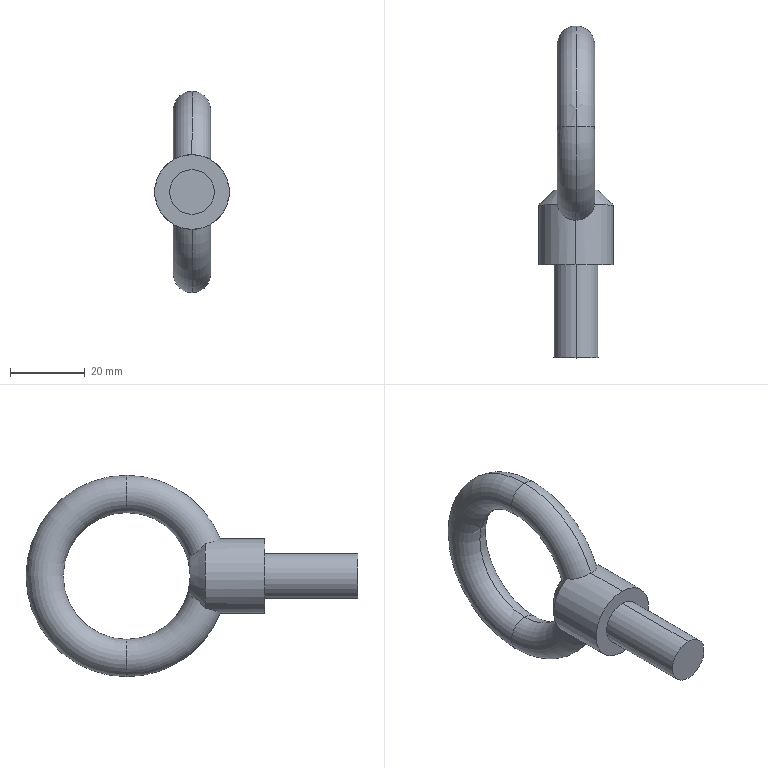Component | SolidWorks | LiftingRingM12-1 | 1 solid | 16 faces | box 20 x 89 x 54 mm | volume 18196 mm3 | torus 6 | cylinder 4 | plane 4 | cone 2 | commonest cylinder face diameters 12 x2 20 x2
STEP:
#1=COLOUR_RGB('',0.7922,0.8196,0.9333);
#2=FILL_AREA_STYLE_COLOUR('',#1);
#3=FILL_AREA_STYLE('',(#2));
#4=SURFACE_STYLE_FILL_AREA(#3);
#5=SURFACE_SIDE_STYLE('',(#4));
#6=SURFACE_STYLE_USAGE(.BOTH.,#5);
#7=PRESENTATION_STYLE_ASSIGNMENT((#6));
#8=CARTESIAN_POINT('',(10.903,79.349,13.168));
#9=VERTEX_POINT('',#8);
#10=CARTESIAN_POINT('',(10.903,79.349,12.775));
#11=VERTEX_POINT('',#10);
#12=CARTESIAN_POINT('',(10.903,79.349,12.971));
#13=DIRECTION('',(0.,1.,0.));
#14=DIRECTION('',(0.,0.,1.));
#15=AXIS2_PLACEMENT_3D('',#12,#13,#14);
#16=CIRCLE('',#15,0.1969);
#17=EDGE_CURVE('',#9,#11,#16,.T.);
#18=ORIENTED_EDGE('',*,*,#17,.F.);
#19=CARTESIAN_POINT('',(10.903,78.361,12.499));
#20=VERTEX_POINT('',#19);
#21=CARTESIAN_POINT('',(10.903,79.349,12.105));
#22=DIRECTION('',(1.,0.,-0.));
#23=DIRECTION('',(0.,0.,-1.));
#24=AXIS2_PLACEMENT_3D('',#21,#22,#23);
#25=CIRCLE('',#24,1.063);
#26=EDGE_CURVE('',#9,#20,#25,.T.);
#27=ORIENTED_EDGE('',*,*,#26,.T.);
#28=CARTESIAN_POINT('',(11.098,78.522,12.447));
#29=VERTEX_POINT('',#28);
#30=CARTESIAN_POINT('',(10.903,78.361,12.499));
#31=CARTESIAN_POINT('',(10.915,78.361,12.499));
#32=CARTESIAN_POINT('',(10.927,78.362,12.498));
#33=CARTESIAN_POINT('',(10.95,78.366,12.496));
#34=CARTESIAN_POINT('',(10.961,78.369,12.495));
#35=CARTESIAN_POINT('',(10.983,78.376,12.491));
#36=CARTESIAN_POINT('',(10.994,78.381,12.489));
#37=CARTESIAN_POINT('',(11.014,78.392,12.483));
#38=CARTESIAN_POINT('',(11.024,78.398,12.48));
#39=CARTESIAN_POINT('',(11.041,78.412,12.474));
#40=CARTESIAN_POINT('',(11.049,78.42,12.471));
#41=CARTESIAN_POINT('',(11.064,78.437,12.465));
#42=CARTESIAN_POINT('',(11.071,78.446,12.462));
#43=CARTESIAN_POINT('',(11.079,78.461,12.458));
#44=CARTESIAN_POINT('',(11.082,78.466,12.456));
#45=CARTESIAN_POINT('',(11.086,78.477,12.454));
#46=CARTESIAN_POINT('',(11.088,78.483,12.453));
#47=CARTESIAN_POINT('',(11.094,78.499,12.45));
#48=CARTESIAN_POINT('',(11.096,78.51,12.448));
#49=CARTESIAN_POINT('',(11.098,78.522,12.447));
#50=B_SPLINE_CURVE_WITH_KNOTS('',3,(#30,#31,#32,#33,#34,#35,#36,#37,#38,#39,#40,#41,#42,#43,#44,#45,#46,#47,#48,#49),.UNSPECIFIED.,.F.,.F.,(4,2,2,2,2,2,2,2,2,4),(0.01123,0.01212,0.01301,0.01389,0.01478,0.01567,0.01656,0.017,0.01744,0.01833),.UNSPECIFIED.);
#51=EDGE_CURVE('',#20,#29,#50,.T.);
#52=ORIENTED_EDGE('',*,*,#51,.T.);
#53=CARTESIAN_POINT('',(11.011,78.68,12.315));
#54=VERTEX_POINT('',#53);
#55=CARTESIAN_POINT('',(11.098,78.522,12.447));
#56=CARTESIAN_POINT('',(11.1,78.534,12.432));
#57=CARTESIAN_POINT('',(11.101,78.547,12.417));
#58=CARTESIAN_POINT('',(11.098,78.567,12.395));
#59=CARTESIAN_POINT('',(11.096,78.574,12.388));
#60=CARTESIAN_POINT('',(11.091,78.588,12.374));
#61=CARTESIAN_POINT('',(11.088,78.595,12.368));
#62=CARTESIAN_POINT('',(11.081,78.609,12.356));
#63=CARTESIAN_POINT('',(11.077,78.616,12.35));
#64=CARTESIAN_POINT('',(11.067,78.63,12.34));
#65=CARTESIAN_POINT('',(11.061,78.636,12.335));
#66=CARTESIAN_POINT('',(11.049,78.65,12.328));
#67=CARTESIAN_POINT('',(11.042,78.656,12.324));
#68=CARTESIAN_POINT('',(11.027,78.669,12.319));
#69=CARTESIAN_POINT('',(11.019,78.674,12.317));
#70=CARTESIAN_POINT('',(11.011,78.68,12.315));
#71=B_SPLINE_CURVE_WITH_KNOTS('',3,(#55,#56,#57,#58,#59,#60,#61,#62,#63,#64,#65,#66,#67,#68,#69,#70),.UNSPECIFIED.,.F.,.F.,(4,2,2,2,2,2,2,4),(0.,0.001504,0.002256,0.003009,0.003761,0.004513,0.005265,0.006017),.UNSPECIFIED.);
#72=EDGE_CURVE('',#29,#54,#71,.T.);
#73=ORIENTED_EDGE('',*,*,#72,.T.);
#74=CARTESIAN_POINT('',(10.903,78.68,12.105));
#75=VERTEX_POINT('',#74);
#76=CARTESIAN_POINT('',(11.011,78.68,12.315));
#77=CARTESIAN_POINT('',(10.995,78.68,12.28));
#78=CARTESIAN_POINT('',(10.977,78.68,12.244));
#79=CARTESIAN_POINT('',(10.95,78.68,12.192));
#80=CARTESIAN_POINT('',(10.941,78.68,12.175));
#81=CARTESIAN_POINT('',(10.922,78.68,12.14));
#82=CARTESIAN_POINT('',(10.913,78.68,12.123));
#83=CARTESIAN_POINT('',(10.903,78.68,12.105));
#84=B_SPLINE_CURVE_WITH_KNOTS('',3,(#76,#77,#78,#79,#80,#81,#82,#83),.UNSPECIFIED.,.F.,.F.,(4,2,2,4),(0.01537,0.01838,0.01989,0.02139),.UNSPECIFIED.);
#85=EDGE_CURVE('',#54,#75,#84,.T.);
#86=ORIENTED_EDGE('',*,*,#85,.T.);
#87=CARTESIAN_POINT('',(10.903,79.349,12.105));
#88=DIRECTION('',(1.,0.,-0.));
#89=DIRECTION('',(0.,0.,-1.));
#90=AXIS2_PLACEMENT_3D('',#87,#88,#89);
#91=CIRCLE('',#90,0.6693);
#92=EDGE_CURVE('',#11,#75,#91,.T.);
#93=ORIENTED_EDGE('',*,*,#92,.F.);
#94=EDGE_LOOP('',(#18,#27,#52,#73,#86,#93));
#95=FACE_OUTER_BOUND('',#94,.T.);
#96=CARTESIAN_POINT('',(10.903,79.349,12.105));
#97=DIRECTION('',(1.,0.,-0.));
#98=DIRECTION('',(0.,0.,1.));
#99=AXIS2_PLACEMENT_3D('',#96,#97,#98);
#100=TOROIDAL_SURFACE('',#99,0.8661,0.1969);
#101=ADVANCED_FACE('',(#95),#100,.T.);
#102=CARTESIAN_POINT('',(10.903,79.349,11.042));
#103=VERTEX_POINT('',#102);
#104=CARTESIAN_POINT('',(10.903,79.349,11.436));
#105=VERTEX_POINT('',#104);
#106=CARTESIAN_POINT('',(10.903,79.349,11.239));
#107=DIRECTION('',(0.,-1.,0.));
#108=DIRECTION('',(0.,0.,-1.));
#109=AXIS2_PLACEMENT_3D('',#106,#107,#108);
#110=CIRCLE('',#109,0.1969);
#111=EDGE_CURVE('',#103,#105,#110,.T.);
#112=ORIENTED_EDGE('',*,*,#111,.F.);
#113=CARTESIAN_POINT('',(10.903,79.349,12.105));
#114=DIRECTION('',(1.,0.,-0.));
#115=DIRECTION('',(0.,0.,-1.));
#116=AXIS2_PLACEMENT_3D('',#113,#114,#115);
#117=CIRCLE('',#116,1.063);
#118=EDGE_CURVE('',#103,#9,#117,.T.);
#119=ORIENTED_EDGE('',*,*,#118,.T.);
#120=ORIENTED_EDGE('',*,*,#17,.T.);
#121=CARTESIAN_POINT('',(10.903,79.349,12.105));
#122=DIRECTION('',(1.,0.,-0.));
#123=DIRECTION('',(0.,0.,-1.));
#124=AXIS2_PLACEMENT_3D('',#121,#122,#123);
#125=CIRCLE('',#124,0.6693);
#126=EDGE_CURVE('',#105,#11,#125,.T.);
#127=ORIENTED_EDGE('',*,*,#126,.F.);
#128=EDGE_LOOP('',(#112,#119,#120,#127));
#129=FACE_OUTER_BOUND('',#128,.T.);
#130=CARTESIAN_POINT('',(10.903,79.349,12.105));
#131=DIRECTION('',(1.,0.,-0.));
#132=DIRECTION('',(0.,0.,1.));
#133=AXIS2_PLACEMENT_3D('',#130,#131,#132);
#134=TOROIDAL_SURFACE('',#133,0.8661,0.1969);
#135=ADVANCED_FACE('',(#129),#134,.T.);
#136=CARTESIAN_POINT('',(11.098,78.522,11.763));
#137=VERTEX_POINT('',#136);
#138=CARTESIAN_POINT('',(10.903,78.361,11.712));
#139=VERTEX_POINT('',#138);
#140=CARTESIAN_POINT('',(11.098,78.522,11.763));
#141=CARTESIAN_POINT('',(11.095,78.499,11.761));
#142=CARTESIAN_POINT('',(11.088,78.477,11.757));
#143=CARTESIAN_POINT('',(11.071,78.446,11.749));
#144=CARTESIAN_POINT('',(11.064,78.437,11.746));
#145=CARTESIAN_POINT('',(11.05,78.42,11.74));
#146=CARTESIAN_POINT('',(11.041,78.412,11.736));
#147=CARTESIAN_POINT('',(11.024,78.398,11.73));
#148=CARTESIAN_POINT('',(11.014,78.392,11.727));
#149=CARTESIAN_POINT('',(10.994,78.381,11.722));
#150=CARTESIAN_POINT('',(10.983,78.376,11.72));
#151=CARTESIAN_POINT('',(10.961,78.369,11.716));
#152=CARTESIAN_POINT('',(10.95,78.366,11.714));
#153=CARTESIAN_POINT('',(10.927,78.362,11.712));
#154=CARTESIAN_POINT('',(10.915,78.361,11.712));
#155=CARTESIAN_POINT('',(10.903,78.361,11.712));
#156=B_SPLINE_CURVE_WITH_KNOTS('',3,(#140,#141,#142,#143,#144,#145,#146,#147,#148,#149,#150,#151,#152,#153,#154,#155),.UNSPECIFIED.,.F.,.F.,(4,2,2,2,2,2,2,4),(0.004137,0.00591,0.006797,0.007684,0.008571,0.009457,0.01034,0.01123),.UNSPECIFIED.);
#157=EDGE_CURVE('',#137,#139,#156,.T.);
#158=ORIENTED_EDGE('',*,*,#157,.T.);
#159=CARTESIAN_POINT('',(10.903,79.349,12.105));
#160=DIRECTION('',(1.,0.,-0.));
#161=DIRECTION('',(0.,0.,-1.));
#162=AXIS2_PLACEMENT_3D('',#159,#160,#161);
#163=CIRCLE('',#162,1.063);
#164=EDGE_CURVE('',#139,#103,#163,.T.);
#165=ORIENTED_EDGE('',*,*,#164,.T.);
#166=ORIENTED_EDGE('',*,*,#111,.T.);
#167=CARTESIAN_POINT('',(10.903,79.349,12.105));
#168=DIRECTION('',(1.,0.,-0.));
#169=DIRECTION('',(0.,0.,-1.));
#170=AXIS2_PLACEMENT_3D('',#167,#168,#169);
#171=CIRCLE('',#170,0.6693);
#172=EDGE_CURVE('',#75,#105,#171,.T.);
#173=ORIENTED_EDGE('',*,*,#172,.F.);
#174=CARTESIAN_POINT('',(11.011,78.68,11.895));
#175=VERTEX_POINT('',#174);
#176=CARTESIAN_POINT('',(10.903,78.68,12.105));
#177=CARTESIAN_POINT('',(10.922,78.68,12.071));
#178=CARTESIAN_POINT('',(10.941,78.68,12.036));
#179=CARTESIAN_POINT('',(10.977,78.68,11.966));
#180=CARTESIAN_POINT('',(10.995,78.68,11.931));
#181=CARTESIAN_POINT('',(11.011,78.68,11.895));
#182=B_SPLINE_CURVE_WITH_KNOTS('',3,(#176,#177,#178,#179,#180,#181),.UNSPECIFIED.,.F.,.F.,(4,2,4),(-0.00002608,0.002971,0.005968),.UNSPECIFIED.);
#183=EDGE_CURVE('',#75,#175,#182,.T.);
#184=ORIENTED_EDGE('',*,*,#183,.T.);
#185=CARTESIAN_POINT('',(11.011,78.68,11.895));
#186=CARTESIAN_POINT('',(11.028,78.669,11.892));
#187=CARTESIAN_POINT('',(11.043,78.657,11.887));
#188=CARTESIAN_POINT('',(11.061,78.637,11.875));
#189=CARTESIAN_POINT('',(11.067,78.63,11.871));
#190=CARTESIAN_POINT('',(11.077,78.616,11.861));
#191=CARTESIAN_POINT('',(11.081,78.609,11.855));
#192=CARTESIAN_POINT('',(11.088,78.595,11.843));
#193=CARTESIAN_POINT('',(11.091,78.588,11.836));
#194=CARTESIAN_POINT('',(11.096,78.574,11.823));
#195=CARTESIAN_POINT('',(11.098,78.567,11.816));
#196=CARTESIAN_POINT('',(11.101,78.547,11.794));
#197=CARTESIAN_POINT('',(11.1,78.534,11.779));
#198=CARTESIAN_POINT('',(11.098,78.522,11.763));
#199=B_SPLINE_CURVE_WITH_KNOTS('',3,(#185,#186,#187,#188,#189,#190,#191,#192,#193,#194,#195,#196,#197,#198),.UNSPECIFIED.,.F.,.F.,(4,2,2,2,2,2,4),(0.,0.001505,0.002258,0.003011,0.003763,0.004516,0.006021),.UNSPECIFIED.);
#200=EDGE_CURVE('',#175,#137,#199,.T.);
#201=ORIENTED_EDGE('',*,*,#200,.T.);
#202=EDGE_LOOP('',(#158,#165,#166,#173,#184,#201));
#203=FACE_OUTER_BOUND('',#202,.T.);
#204=CARTESIAN_POINT('',(10.903,79.349,12.105));
#205=DIRECTION('',(1.,0.,-0.));
#206=DIRECTION('',(0.,0.,1.));
#207=AXIS2_PLACEMENT_3D('',#204,#205,#206);
#208=TOROIDAL_SURFACE('',#207,0.8661,0.1969);
#209=ADVANCED_FACE('',(#203),#208,.T.);
#210=CARTESIAN_POINT('',(10.903,76.908,11.869));
#211=VERTEX_POINT('',#210);
#212=CARTESIAN_POINT('',(10.903,76.908,12.341));
#213=VERTEX_POINT('',#212);
#214=CARTESIAN_POINT('',(10.903,76.908,12.105));
#215=DIRECTION('',(0.,-1.,0.));
#216=DIRECTION('',(0.,0.,-1.));
#217=AXIS2_PLACEMENT_3D('',#214,#215,#216);
#218=CIRCLE('',#217,0.2362);
#219=EDGE_CURVE('',#211,#213,#218,.T.);
#220=ORIENTED_EDGE('',*,*,#219,.F.);
#221=CARTESIAN_POINT('',(10.903,77.892,11.869));
#222=VERTEX_POINT('',#221);
#223=CARTESIAN_POINT('',(10.903,76.908,11.869));
#224=DIRECTION('',(0.,1.,0.));
#225=VECTOR('',#224,39.37);
#226=LINE('',#223,#225);
#227=EDGE_CURVE('',#211,#222,#226,.T.);
#228=ORIENTED_EDGE('',*,*,#227,.T.);
#229=CARTESIAN_POINT('',(10.903,77.892,12.341));
#230=VERTEX_POINT('',#229);
#231=CARTESIAN_POINT('',(10.903,77.892,12.105));
#232=DIRECTION('',(0.,-1.,0.));
#233=DIRECTION('',(0.,0.,-1.));
#234=AXIS2_PLACEMENT_3D('',#231,#232,#233);
#235=CIRCLE('',#234,0.2362);
#236=EDGE_CURVE('',#222,#230,#235,.T.);
#237=ORIENTED_EDGE('',*,*,#236,.T.);
#238=CARTESIAN_POINT('',(10.903,76.908,12.341));
#239=DIRECTION('',(0.,1.,0.));
#240=VECTOR('',#239,39.37);
#241=LINE('',#238,#240);
#242=EDGE_CURVE('',#213,#230,#241,.T.);
#243=ORIENTED_EDGE('',*,*,#242,.F.);
#244=EDGE_LOOP('',(#220,#228,#237,#243));
#245=FACE_OUTER_BOUND('',#244,.T.);
#246=CARTESIAN_POINT('',(10.903,76.908,12.105));
#247=DIRECTION('',(0.,1.,0.));
#248=DIRECTION('',(0.,0.,1.));
#249=AXIS2_PLACEMENT_3D('',#246,#247,#248);
#250=CYLINDRICAL_SURFACE('',#249,0.2362);
#251=ADVANCED_FACE('',(#245),#250,.T.);
#252=ORIENTED_EDGE('',*,*,#164,.F.);
#253=CARTESIAN_POINT('',(10.708,78.522,11.763));
#254=VERTEX_POINT('',#253);
#255=CARTESIAN_POINT('',(10.903,78.361,11.712));
#256=CARTESIAN_POINT('',(10.891,78.361,11.712));
#257=CARTESIAN_POINT('',(10.88,78.362,11.712));
#258=CARTESIAN_POINT('',(10.857,78.366,11.714));
#259=CARTESIAN_POINT('',(10.845,78.369,11.716));
#260=CARTESIAN_POINT('',(10.823,78.376,11.72));
#261=CARTESIAN_POINT('',(10.813,78.381,11.722));
#262=CARTESIAN_POINT('',(10.792,78.392,11.727));
#263=CARTESIAN_POINT('',(10.783,78.398,11.73));
#264=CARTESIAN_POINT('',(10.765,78.412,11.736));
#265=CARTESIAN_POINT('',(10.757,78.42,11.74));
#266=CARTESIAN_POINT('',(10.742,78.437,11.746));
#267=CARTESIAN_POINT('',(10.736,78.446,11.749));
#268=CARTESIAN_POINT('',(10.727,78.461,11.753));
#269=CARTESIAN_POINT('',(10.725,78.466,11.754));
#270=CARTESIAN_POINT('',(10.72,78.477,11.757));
#271=CARTESIAN_POINT('',(10.718,78.483,11.758));
#272=CARTESIAN_POINT('',(10.713,78.499,11.761));
#273=CARTESIAN_POINT('',(10.71,78.51,11.762));
#274=CARTESIAN_POINT('',(10.708,78.522,11.763));
#275=B_SPLINE_CURVE_WITH_KNOTS('',3,(#255,#256,#257,#258,#259,#260,#261,#262,#263,#264,#265,#266,#267,#268,#269,#270,#271,#272,#273,#274),.UNSPECIFIED.,.F.,.F.,(4,2,2,2,2,2,2,2,2,4),(0.01123,0.01212,0.01301,0.01389,0.01478,0.01567,0.01656,0.017,0.01744,0.01833),.UNSPECIFIED.);
#276=EDGE_CURVE('',#139,#254,#275,.T.);
#277=ORIENTED_EDGE('',*,*,#276,.T.);
#278=CARTESIAN_POINT('',(10.795,78.68,11.895));
#279=VERTEX_POINT('',#278);
#280=CARTESIAN_POINT('',(10.708,78.522,11.763));
#281=CARTESIAN_POINT('',(10.706,78.534,11.779));
#282=CARTESIAN_POINT('',(10.706,78.547,11.794));
#283=CARTESIAN_POINT('',(10.709,78.567,11.816));
#284=CARTESIAN_POINT('',(10.711,78.574,11.823));
#285=CARTESIAN_POINT('',(10.715,78.588,11.836));
#286=CARTESIAN_POINT('',(10.718,78.595,11.843));
#287=CARTESIAN_POINT('',(10.725,78.609,11.855));
#288=CARTESIAN_POINT('',(10.73,78.616,11.86));
#289=CARTESIAN_POINT('',(10.739,78.63,11.871));
#290=CARTESIAN_POINT('',(10.745,78.636,11.875));
#291=CARTESIAN_POINT('',(10.757,78.65,11.883));
#292=CARTESIAN_POINT('',(10.764,78.656,11.886));
#293=CARTESIAN_POINT('',(10.779,78.669,11.891));
#294=CARTESIAN_POINT('',(10.787,78.674,11.894));
#295=CARTESIAN_POINT('',(10.795,78.68,11.895));
#296=B_SPLINE_CURVE_WITH_KNOTS('',3,(#280,#281,#282,#283,#284,#285,#286,#287,#288,#289,#290,#291,#292,#293,#294,#295),.UNSPECIFIED.,.F.,.F.,(4,2,2,2,2,2,2,4),(0.,0.001504,0.002256,0.003009,0.003761,0.004513,0.005265,0.006017),.UNSPECIFIED.);
#297=EDGE_CURVE('',#254,#279,#296,.T.);
#298=ORIENTED_EDGE('',*,*,#297,.T.);
#299=CARTESIAN_POINT('',(10.795,78.68,11.895));
#300=CARTESIAN_POINT('',(10.812,78.68,11.931));
#301=CARTESIAN_POINT('',(10.829,78.68,11.966));
#302=CARTESIAN_POINT('',(10.857,78.68,12.019));
#303=CARTESIAN_POINT('',(10.866,78.68,12.036));
#304=CARTESIAN_POINT('',(10.884,78.68,12.071));
#305=CARTESIAN_POINT('',(10.894,78.68,12.088));
#306=CARTESIAN_POINT('',(10.903,78.68,12.105));
#307=B_SPLINE_CURVE_WITH_KNOTS('',3,(#299,#300,#301,#302,#303,#304,#305,#306),.UNSPECIFIED.,.F.,.F.,(4,2,2,4),(0.01537,0.01838,0.01989,0.02139),.UNSPECIFIED.);
#308=EDGE_CURVE('',#279,#75,#307,.T.);
#309=ORIENTED_EDGE('',*,*,#308,.T.);
#310=ORIENTED_EDGE('',*,*,#172,.T.);
#311=CARTESIAN_POINT('',(10.903,79.349,11.239));
#312=DIRECTION('',(0.,-1.,0.));
#313=DIRECTION('',(0.,0.,-1.));
#314=AXIS2_PLACEMENT_3D('',#311,#312,#313);
#315=CIRCLE('',#314,0.1969);
#316=EDGE_CURVE('',#105,#103,#315,.T.);
#317=ORIENTED_EDGE('',*,*,#316,.T.);
#318=EDGE_LOOP('',(#252,#277,#298,#309,#310,#317));
#319=FACE_OUTER_BOUND('',#318,.T.);
#320=CARTESIAN_POINT('',(10.903,79.349,12.105));
#321=DIRECTION('',(1.,0.,-0.));
#322=DIRECTION('',(0.,0.,1.));
#323=AXIS2_PLACEMENT_3D('',#320,#321,#322);
#324=TOROIDAL_SURFACE('',#323,0.8661,0.1969);
#325=ADVANCED_FACE('',(#319),#324,.T.);
#326=ORIENTED_EDGE('',*,*,#118,.F.);
#327=ORIENTED_EDGE('',*,*,#316,.F.);
#328=ORIENTED_EDGE('',*,*,#126,.T.);
#329=CARTESIAN_POINT('',(10.903,79.349,12.971));
#330=DIRECTION('',(0.,1.,0.));
#331=DIRECTION('',(0.,0.,1.));
#332=AXIS2_PLACEMENT_3D('',#329,#330,#331);
#333=CIRCLE('',#332,0.1969);
#334=EDGE_CURVE('',#11,#9,#333,.T.);
#335=ORIENTED_EDGE('',*,*,#334,.T.);
#336=EDGE_LOOP('',(#326,#327,#328,#335));
#337=FACE_OUTER_BOUND('',#336,.T.);
#338=CARTESIAN_POINT('',(10.903,79.349,12.105));
#339=DIRECTION('',(1.,0.,-0.));
#340=DIRECTION('',(0.,0.,1.));
#341=AXIS2_PLACEMENT_3D('',#338,#339,#340);
#342=TOROIDAL_SURFACE('',#341,0.8661,0.1969);
#343=ADVANCED_FACE('',(#337),#342,.T.);
#344=CARTESIAN_POINT('',(10.903,77.892,11.712));
#345=VERTEX_POINT('',#344);
#346=CARTESIAN_POINT('',(10.903,77.892,12.499));
#347=VERTEX_POINT('',#346);
#348=CARTESIAN_POINT('',(10.903,77.892,12.105));
#349=DIRECTION('',(0.,-1.,0.));
#350=DIRECTION('',(0.,0.,-1.));
#351=AXIS2_PLACEMENT_3D('',#348,#349,#350);
#352=CIRCLE('',#351,0.3937);
#353=EDGE_CURVE('',#345,#347,#352,.T.);
#354=ORIENTED_EDGE('',*,*,#353,.F.);
#355=CARTESIAN_POINT('',(10.903,77.892,11.712));
#356=DIRECTION('',(0.,1.,0.));
#357=VECTOR('',#356,39.37);
#358=LINE('',#355,#357);
#359=EDGE_CURVE('',#345,#139,#358,.T.);
#360=ORIENTED_EDGE('',*,*,#359,.T.);
#361=ORIENTED_EDGE('',*,*,#157,.F.);
#362=CARTESIAN_POINT('',(10.903,78.522,12.105));
#363=DIRECTION('',(0.,-1.,0.));
#364=DIRECTION('',(0.,0.,-1.));
#365=AXIS2_PLACEMENT_3D('',#362,#363,#364);
#366=CIRCLE('',#365,0.3937);
#367=EDGE_CURVE('',#137,#29,#366,.T.);
#368=ORIENTED_EDGE('',*,*,#367,.T.);
#369=ORIENTED_EDGE('',*,*,#51,.F.);
#370=CARTESIAN_POINT('',(10.903,77.892,12.499));
#371=DIRECTION('',(0.,1.,0.));
#372=VECTOR('',#371,39.37);
#373=LINE('',#370,#372);
#374=EDGE_CURVE('',#347,#20,#373,.T.);
#375=ORIENTED_EDGE('',*,*,#374,.F.);
#376=EDGE_LOOP('',(#354,#360,#361,#368,#369,#375));
#377=FACE_OUTER_BOUND('',#376,.T.);
#378=CARTESIAN_POINT('',(10.903,77.892,12.105));
#379=DIRECTION('',(0.,1.,0.));
#380=DIRECTION('',(0.,0.,1.));
#381=AXIS2_PLACEMENT_3D('',#378,#379,#380);
#382=CYLINDRICAL_SURFACE('',#381,0.3937);
#383=ADVANCED_FACE('',(#377),#382,.T.);
#384=CARTESIAN_POINT('',(10.903,77.892,12.105));
#385=DIRECTION('',(0.,-1.,0.));
#386=DIRECTION('',(0.,0.,-1.));
#387=AXIS2_PLACEMENT_3D('',#384,#385,#386);
#388=CIRCLE('',#387,0.3937);
#389=EDGE_CURVE('',#347,#345,#388,.T.);
#390=ORIENTED_EDGE('',*,*,#389,.T.);
#391=ORIENTED_EDGE('',*,*,#353,.T.);
#392=EDGE_LOOP('',(#390,#391));
#393=FACE_OUTER_BOUND('',#392,.T.);
#394=CARTESIAN_POINT('',(10.903,77.892,12.105));
#395=DIRECTION('',(0.,-1.,0.));
#396=DIRECTION('',(0.,0.,-1.));
#397=AXIS2_PLACEMENT_3D('',#394,#395,#396);
#398=CIRCLE('',#397,0.2362);
#399=EDGE_CURVE('',#230,#222,#398,.T.);
#400=ORIENTED_EDGE('',*,*,#399,.F.);
#401=ORIENTED_EDGE('',*,*,#236,.F.);
#402=EDGE_LOOP('',(#400,#401));
#403=FACE_BOUND('',#402,.T.);
#404=CARTESIAN_POINT('',(10.903,77.892,12.105));
#405=DIRECTION('',(0.,-1.,0.));
#406=DIRECTION('',(-0.,0.,-1.));
#407=AXIS2_PLACEMENT_3D('',#404,#405,#406);
#408=PLANE('',#407);
#409=ADVANCED_FACE('',(#393,#403),#408,.T.);
#410=ORIENTED_EDGE('',*,*,#308,.F.);
#411=CARTESIAN_POINT('',(10.795,78.68,12.315));
#412=VERTEX_POINT('',#411);
#413=CARTESIAN_POINT('',(10.903,78.68,12.105));
#414=DIRECTION('',(0.,1.,0.));
#415=DIRECTION('',(0.,0.,-1.));
#416=AXIS2_PLACEMENT_3D('',#413,#414,#415);
#417=CIRCLE('',#416,0.2362);
#418=EDGE_CURVE('',#279,#412,#417,.T.);
#419=ORIENTED_EDGE('',*,*,#418,.T.);
#420=CARTESIAN_POINT('',(10.903,78.68,12.105));
#421=CARTESIAN_POINT('',(10.884,78.68,12.14));
#422=CARTESIAN_POINT('',(10.866,78.68,12.175));
#423=CARTESIAN_POINT('',(10.829,78.68,12.244));
#424=CARTESIAN_POINT('',(10.812,78.68,12.28));
#425=CARTESIAN_POINT('',(10.795,78.68,12.315));
#426=B_SPLINE_CURVE_WITH_KNOTS('',3,(#420,#421,#422,#423,#424,#425),.UNSPECIFIED.,.F.,.F.,(4,2,4),(-0.00002608,0.002971,0.005968),.UNSPECIFIED.);
#427=EDGE_CURVE('',#75,#412,#426,.T.);
#428=ORIENTED_EDGE('',*,*,#427,.F.);
#429=EDGE_LOOP('',(#410,#419,#428));
#430=FACE_OUTER_BOUND('',#429,.T.);
#431=CARTESIAN_POINT('',(10.903,78.68,12.105));
#432=DIRECTION('',(0.,-1.,0.));
#433=DIRECTION('',(-0.,0.,-1.));
#434=AXIS2_PLACEMENT_3D('',#431,#432,#433);
#435=PLANE('',#434);
#436=ADVANCED_FACE('',(#430),#435,.F.);
#437=ORIENTED_EDGE('',*,*,#359,.F.);
#438=ORIENTED_EDGE('',*,*,#389,.F.);
#439=ORIENTED_EDGE('',*,*,#374,.T.);
#440=CARTESIAN_POINT('',(10.708,78.522,12.447));
#441=VERTEX_POINT('',#440);
#442=CARTESIAN_POINT('',(10.708,78.522,12.447));
#443=CARTESIAN_POINT('',(10.712,78.499,12.449));
#444=CARTESIAN_POINT('',(10.719,78.477,12.453));
#445=CARTESIAN_POINT('',(10.736,78.446,12.462));
#446=CARTESIAN_POINT('',(10.742,78.437,12.465));
#447=CARTESIAN_POINT('',(10.757,78.42,12.471));
#448=CARTESIAN_POINT('',(10.765,78.412,12.474));
#449=CARTESIAN_POINT('',(10.783,78.398,12.48));
#450=CARTESIAN_POINT('',(10.792,78.392,12.483));
#451=CARTESIAN_POINT('',(10.813,78.381,12.489));
#452=CARTESIAN_POINT('',(10.823,78.376,12.491));
#453=CARTESIAN_POINT('',(10.845,78.369,12.495));
#454=CARTESIAN_POINT('',(10.856,78.366,12.496));
#455=CARTESIAN_POINT('',(10.88,78.362,12.498));
#456=CARTESIAN_POINT('',(10.891,78.361,12.499));
#457=CARTESIAN_POINT('',(10.903,78.361,12.499));
#458=B_SPLINE_CURVE_WITH_KNOTS('',3,(#442,#443,#444,#445,#446,#447,#448,#449,#450,#451,#452,#453,#454,#455,#456,#457),.UNSPECIFIED.,.F.,.F.,(4,2,2,2,2,2,2,4),(0.004137,0.00591,0.006797,0.007684,0.008571,0.009457,0.01034,0.01123),.UNSPECIFIED.);
#459=EDGE_CURVE('',#441,#20,#458,.T.);
#460=ORIENTED_EDGE('',*,*,#459,.F.);
#461=CARTESIAN_POINT('',(10.903,78.522,12.105));
#462=DIRECTION('',(0.,-1.,0.));
#463=DIRECTION('',(0.,0.,-1.));
#464=AXIS2_PLACEMENT_3D('',#461,#462,#463);
#465=CIRCLE('',#464,0.3937);
#466=EDGE_CURVE('',#441,#254,#465,.T.);
#467=ORIENTED_EDGE('',*,*,#466,.T.);
#468=ORIENTED_EDGE('',*,*,#276,.F.);
#469=EDGE_LOOP('',(#437,#438,#439,#460,#467,#468));
#470=FACE_OUTER_BOUND('',#469,.T.);
#471=CARTESIAN_POINT('',(10.903,77.892,12.105));
#472=DIRECTION('',(0.,1.,0.));
#473=DIRECTION('',(0.,0.,1.));
#474=AXIS2_PLACEMENT_3D('',#471,#472,#473);
#475=CYLINDRICAL_SURFACE('',#474,0.3937);
#476=ADVANCED_FACE('',(#470),#475,.T.);
#477=ORIENTED_EDGE('',*,*,#85,.F.);
#478=CARTESIAN_POINT('',(10.903,78.68,12.105));
#479=DIRECTION('',(0.,1.,0.));
#480=DIRECTION('',(0.,0.,-1.));
#481=AXIS2_PLACEMENT_3D('',#478,#479,#480);
#482=CIRCLE('',#481,0.2362);
#483=EDGE_CURVE('',#54,#175,#482,.T.);
#484=ORIENTED_EDGE('',*,*,#483,.T.);
#485=ORIENTED_EDGE('',*,*,#183,.F.);
#486=EDGE_LOOP('',(#477,#484,#485));
#487=FACE_OUTER_BOUND('',#486,.T.);
#488=CARTESIAN_POINT('',(10.903,78.68,12.105));
#489=DIRECTION('',(0.,-1.,0.));
#490=DIRECTION('',(-0.,0.,-1.));
#491=AXIS2_PLACEMENT_3D('',#488,#489,#490);
#492=PLANE('',#491);
#493=ADVANCED_FACE('',(#487),#492,.F.);
#494=ORIENTED_EDGE('',*,*,#26,.F.);
#495=ORIENTED_EDGE('',*,*,#334,.F.);
#496=ORIENTED_EDGE('',*,*,#92,.T.);
#497=ORIENTED_EDGE('',*,*,#427,.T.);
#498=CARTESIAN_POINT('',(10.795,78.68,12.315));
#499=CARTESIAN_POINT('',(10.779,78.669,12.319));
#500=CARTESIAN_POINT('',(10.764,78.657,12.324));
#501=CARTESIAN_POINT('',(10.745,78.637,12.335));
#502=CARTESIAN_POINT('',(10.739,78.63,12.34));
#503=CARTESIAN_POINT('',(10.73,78.616,12.35));
#504=CARTESIAN_POINT('',(10.725,78.609,12.356));
#505=CARTESIAN_POINT('',(10.718,78.595,12.368));
#506=CARTESIAN_POINT('',(10.715,78.588,12.374));
#507=CARTESIAN_POINT('',(10.711,78.574,12.388));
#508=CARTESIAN_POINT('',(10.709,78.567,12.395));
#509=CARTESIAN_POINT('',(10.706,78.547,12.417));
#510=CARTESIAN_POINT('',(10.706,78.534,12.432));
#511=CARTESIAN_POINT('',(10.708,78.522,12.447));
#512=B_SPLINE_CURVE_WITH_KNOTS('',3,(#498,#499,#500,#501,#502,#503,#504,#505,#506,#507,#508,#509,#510,#511),.UNSPECIFIED.,.F.,.F.,(4,2,2,2,2,2,4),(0.,0.001505,0.002258,0.003011,0.003763,0.004516,0.006021),.UNSPECIFIED.);
#513=EDGE_CURVE('',#412,#441,#512,.T.);
#514=ORIENTED_EDGE('',*,*,#513,.T.);
#515=ORIENTED_EDGE('',*,*,#459,.T.);
#516=EDGE_LOOP('',(#494,#495,#496,#497,#514,#515));
#517=FACE_OUTER_BOUND('',#516,.T.);
#518=CARTESIAN_POINT('',(10.903,79.349,12.105));
#519=DIRECTION('',(1.,0.,-0.));
#520=DIRECTION('',(0.,0.,1.));
#521=AXIS2_PLACEMENT_3D('',#518,#519,#520);
#522=TOROIDAL_SURFACE('',#521,0.8661,0.1969);
#523=ADVANCED_FACE('',(#517),#522,.T.);
#524=ORIENTED_EDGE('',*,*,#227,.F.);
#525=CARTESIAN_POINT('',(10.903,76.908,12.105));
#526=DIRECTION('',(0.,-1.,0.));
#527=DIRECTION('',(0.,0.,-1.));
#528=AXIS2_PLACEMENT_3D('',#525,#526,#527);
#529=CIRCLE('',#528,0.2362);
#530=EDGE_CURVE('',#213,#211,#529,.T.);
#531=ORIENTED_EDGE('',*,*,#530,.F.);
#532=ORIENTED_EDGE('',*,*,#242,.T.);
#533=ORIENTED_EDGE('',*,*,#399,.T.);
#534=EDGE_LOOP('',(#524,#531,#532,#533));
#535=FACE_OUTER_BOUND('',#534,.T.);
#536=CARTESIAN_POINT('',(10.903,76.908,12.105));
#537=DIRECTION('',(0.,1.,0.));
#538=DIRECTION('',(0.,0.,1.));
#539=AXIS2_PLACEMENT_3D('',#536,#537,#538);
#540=CYLINDRICAL_SURFACE('',#539,0.2362);
#541=ADVANCED_FACE('',(#535),#540,.T.);
#542=ORIENTED_EDGE('',*,*,#530,.T.);
#543=ORIENTED_EDGE('',*,*,#219,.T.);
#544=EDGE_LOOP('',(#542,#543));
#545=FACE_OUTER_BOUND('',#544,.T.);
#546=CARTESIAN_POINT('',(10.903,76.908,12.105));
#547=DIRECTION('',(0.,-1.,0.));
#548=DIRECTION('',(-0.,0.,-1.));
#549=AXIS2_PLACEMENT_3D('',#546,#547,#548);
#550=PLANE('',#549);
#551=ADVANCED_FACE('',(#545),#550,.T.);
#552=ORIENTED_EDGE('',*,*,#513,.F.);
#553=ORIENTED_EDGE('',*,*,#418,.F.);
#554=ORIENTED_EDGE('',*,*,#297,.F.);
#555=ORIENTED_EDGE('',*,*,#466,.F.);
#556=EDGE_LOOP('',(#552,#553,#554,#555));
#557=FACE_OUTER_BOUND('',#556,.T.);
#558=CARTESIAN_POINT('',(10.903,78.522,12.105));
#559=DIRECTION('',(0.,-1.,0.));
#560=DIRECTION('',(0.,0.,-1.));
#561=AXIS2_PLACEMENT_3D('',#558,#559,#560);
#562=CONICAL_SURFACE('',#561,0.3937,0.7854);
#563=ADVANCED_FACE('',(#557),#562,.T.);
#564=ORIENTED_EDGE('',*,*,#200,.F.);
#565=ORIENTED_EDGE('',*,*,#483,.F.);
#566=ORIENTED_EDGE('',*,*,#72,.F.);
#567=ORIENTED_EDGE('',*,*,#367,.F.);
#568=EDGE_LOOP('',(#564,#565,#566,#567));
#569=FACE_OUTER_BOUND('',#568,.T.);
#570=CARTESIAN_POINT('',(10.903,78.522,12.105));
#571=DIRECTION('',(0.,-1.,0.));
#572=DIRECTION('',(0.,0.,-1.));
#573=AXIS2_PLACEMENT_3D('',#570,#571,#572);
#574=CONICAL_SURFACE('',#573,0.3937,0.7854);
#575=ADVANCED_FACE('',(#569),#574,.T.);
#576=CLOSED_SHELL('',(#101,#135,#209,#251,#325,#343,#383,#409,#436,#476,#493,#523,#541,#551,#563,#575));
#577=MANIFOLD_SOLID_BREP('',#576);
#578=STYLED_ITEM('',(#7),#577);
#579=(LENGTH_UNIT()NAMED_UNIT(*)SI_UNIT($,.METRE.));
#580=LENGTH_MEASURE_WITH_UNIT(LENGTH_MEASURE(0.0254),#579);
#581=DIMENSIONAL_EXPONENTS(1.,0.,0.,0.,0.,0.,0.);
#582=(CONVERSION_BASED_UNIT('',#580)LENGTH_UNIT()NAMED_UNIT(#581));
#583=UNCERTAINTY_MEASURE_WITH_UNIT(LENGTH_MEASURE(0.00001),#582,'','');
#584=(NAMED_UNIT(*)PLANE_ANGLE_UNIT()SI_UNIT($,.RADIAN.));
#585=(NAMED_UNIT(*)SI_UNIT($,.STERADIAN.)SOLID_ANGLE_UNIT());
#586=(GEOMETRIC_REPRESENTATION_CONTEXT(3)GLOBAL_UNCERTAINTY_ASSIGNED_CONTEXT((#583))GLOBAL_UNIT_ASSIGNED_CONTEXT((#582,#584,#585))REPRESENTATION_CONTEXT('',''));
#587=MECHANICAL_DESIGN_GEOMETRIC_PRESENTATION_REPRESENTATION('',(#578),#586);
#588=PRESENTATION_LAYER_ASSIGNMENT('','',(#578));
#589=CARTESIAN_POINT('',(0.,0.,0.));
#590=DIRECTION('',(0.,0.,1.));
#591=DIRECTION('',(1.,0.,0.));
#592=AXIS2_PLACEMENT_3D('',#589,#590,#591);
#593=(LENGTH_UNIT()NAMED_UNIT(*)SI_UNIT($,.METRE.));
#594=LENGTH_MEASURE_WITH_UNIT(LENGTH_MEASURE(0.0254),#593);
#595=DIMENSIONAL_EXPONENTS(1.,0.,0.,0.,0.,0.,0.);
#596=(CONVERSION_BASED_UNIT('',#594)LENGTH_UNIT()NAMED_UNIT(#595));
#597=UNCERTAINTY_MEASURE_WITH_UNIT(LENGTH_MEASURE(0.00001),#596,'','');
#598=(NAMED_UNIT(*)PLANE_ANGLE_UNIT()SI_UNIT($,.RADIAN.));
#599=(NAMED_UNIT(*)SI_UNIT($,.STERADIAN.)SOLID_ANGLE_UNIT());
#600=(GEOMETRIC_REPRESENTATION_CONTEXT(3)GLOBAL_UNCERTAINTY_ASSIGNED_CONTEXT((#597))GLOBAL_UNIT_ASSIGNED_CONTEXT((#596,#598,#599))REPRESENTATION_CONTEXT('',''));
#601=ADVANCED_BREP_SHAPE_REPRESENTATION('',(#577,#592),#600);